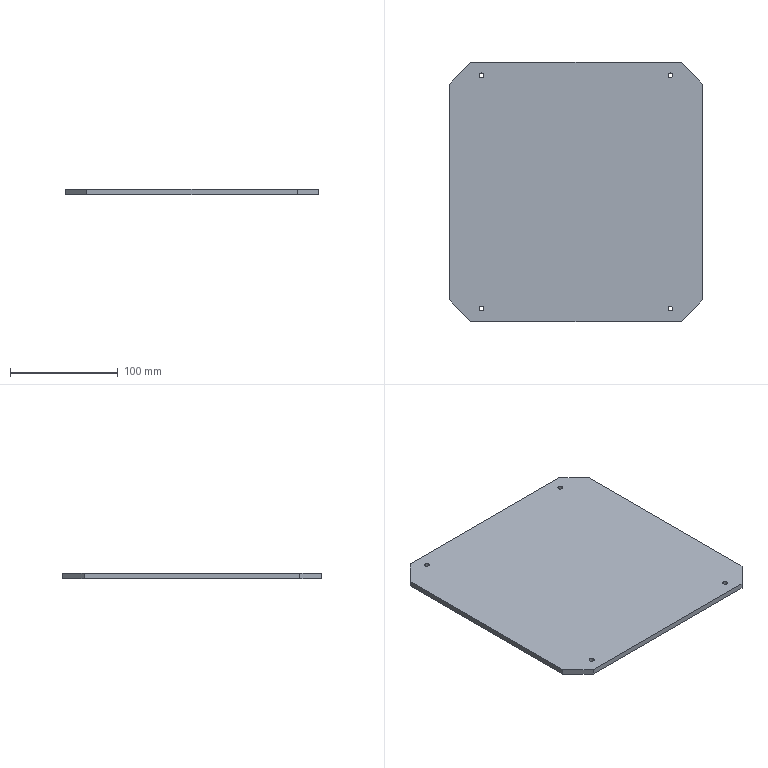CAM job | Mastercam | mm | 5 operations | part box 235 x 240 x 5
1. Contour (Ramp) | 12 - 12 平铣刀
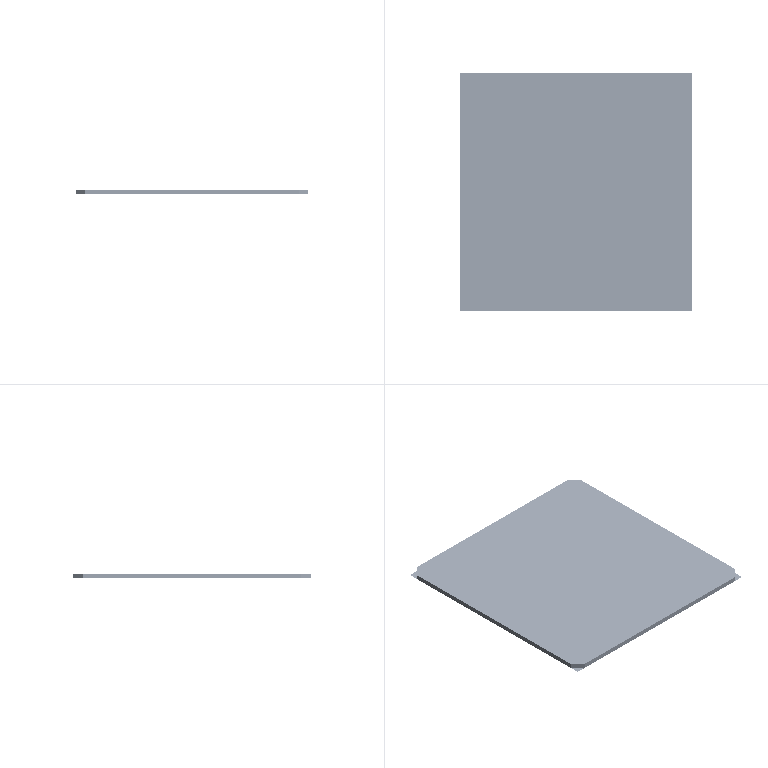2. Contour (Ramp) | 12 - 12 平铣刀
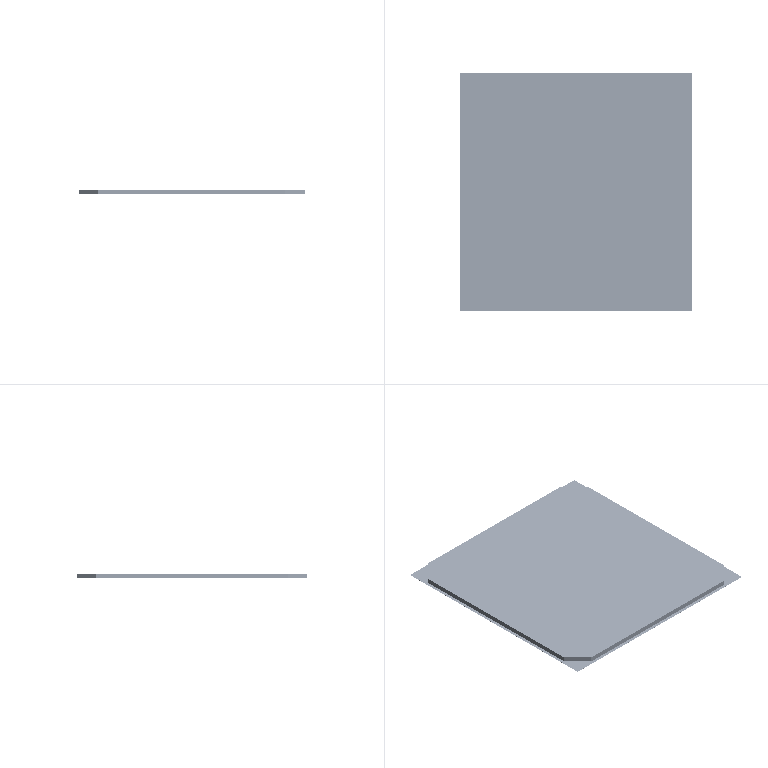3. Contour (2D) | 12 - 12 平铣刀
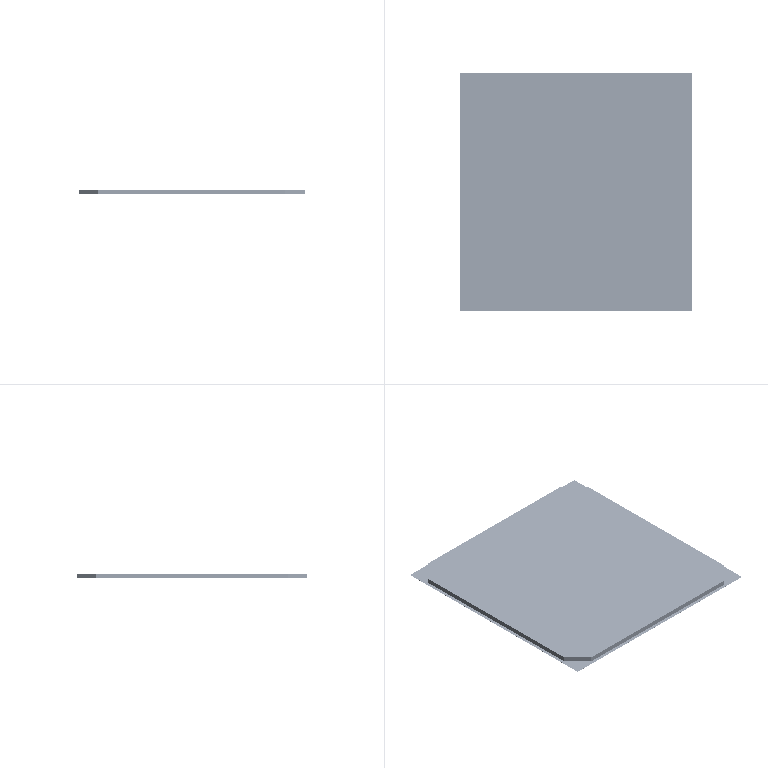4. Drill/Counterbore | 7 - 4 倒角刀
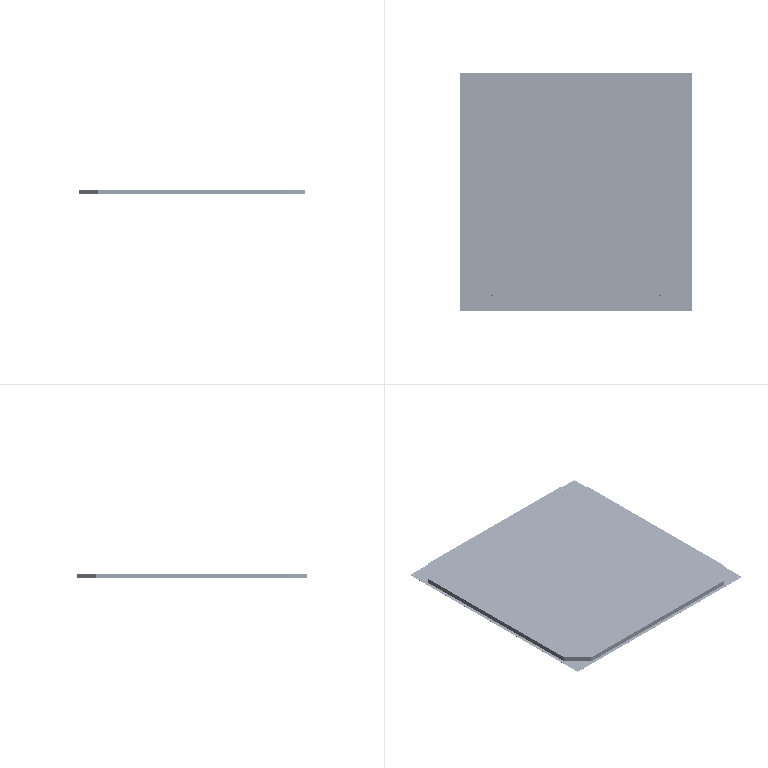5. Contour (2D chamfer) | 7 - 4 倒角刀